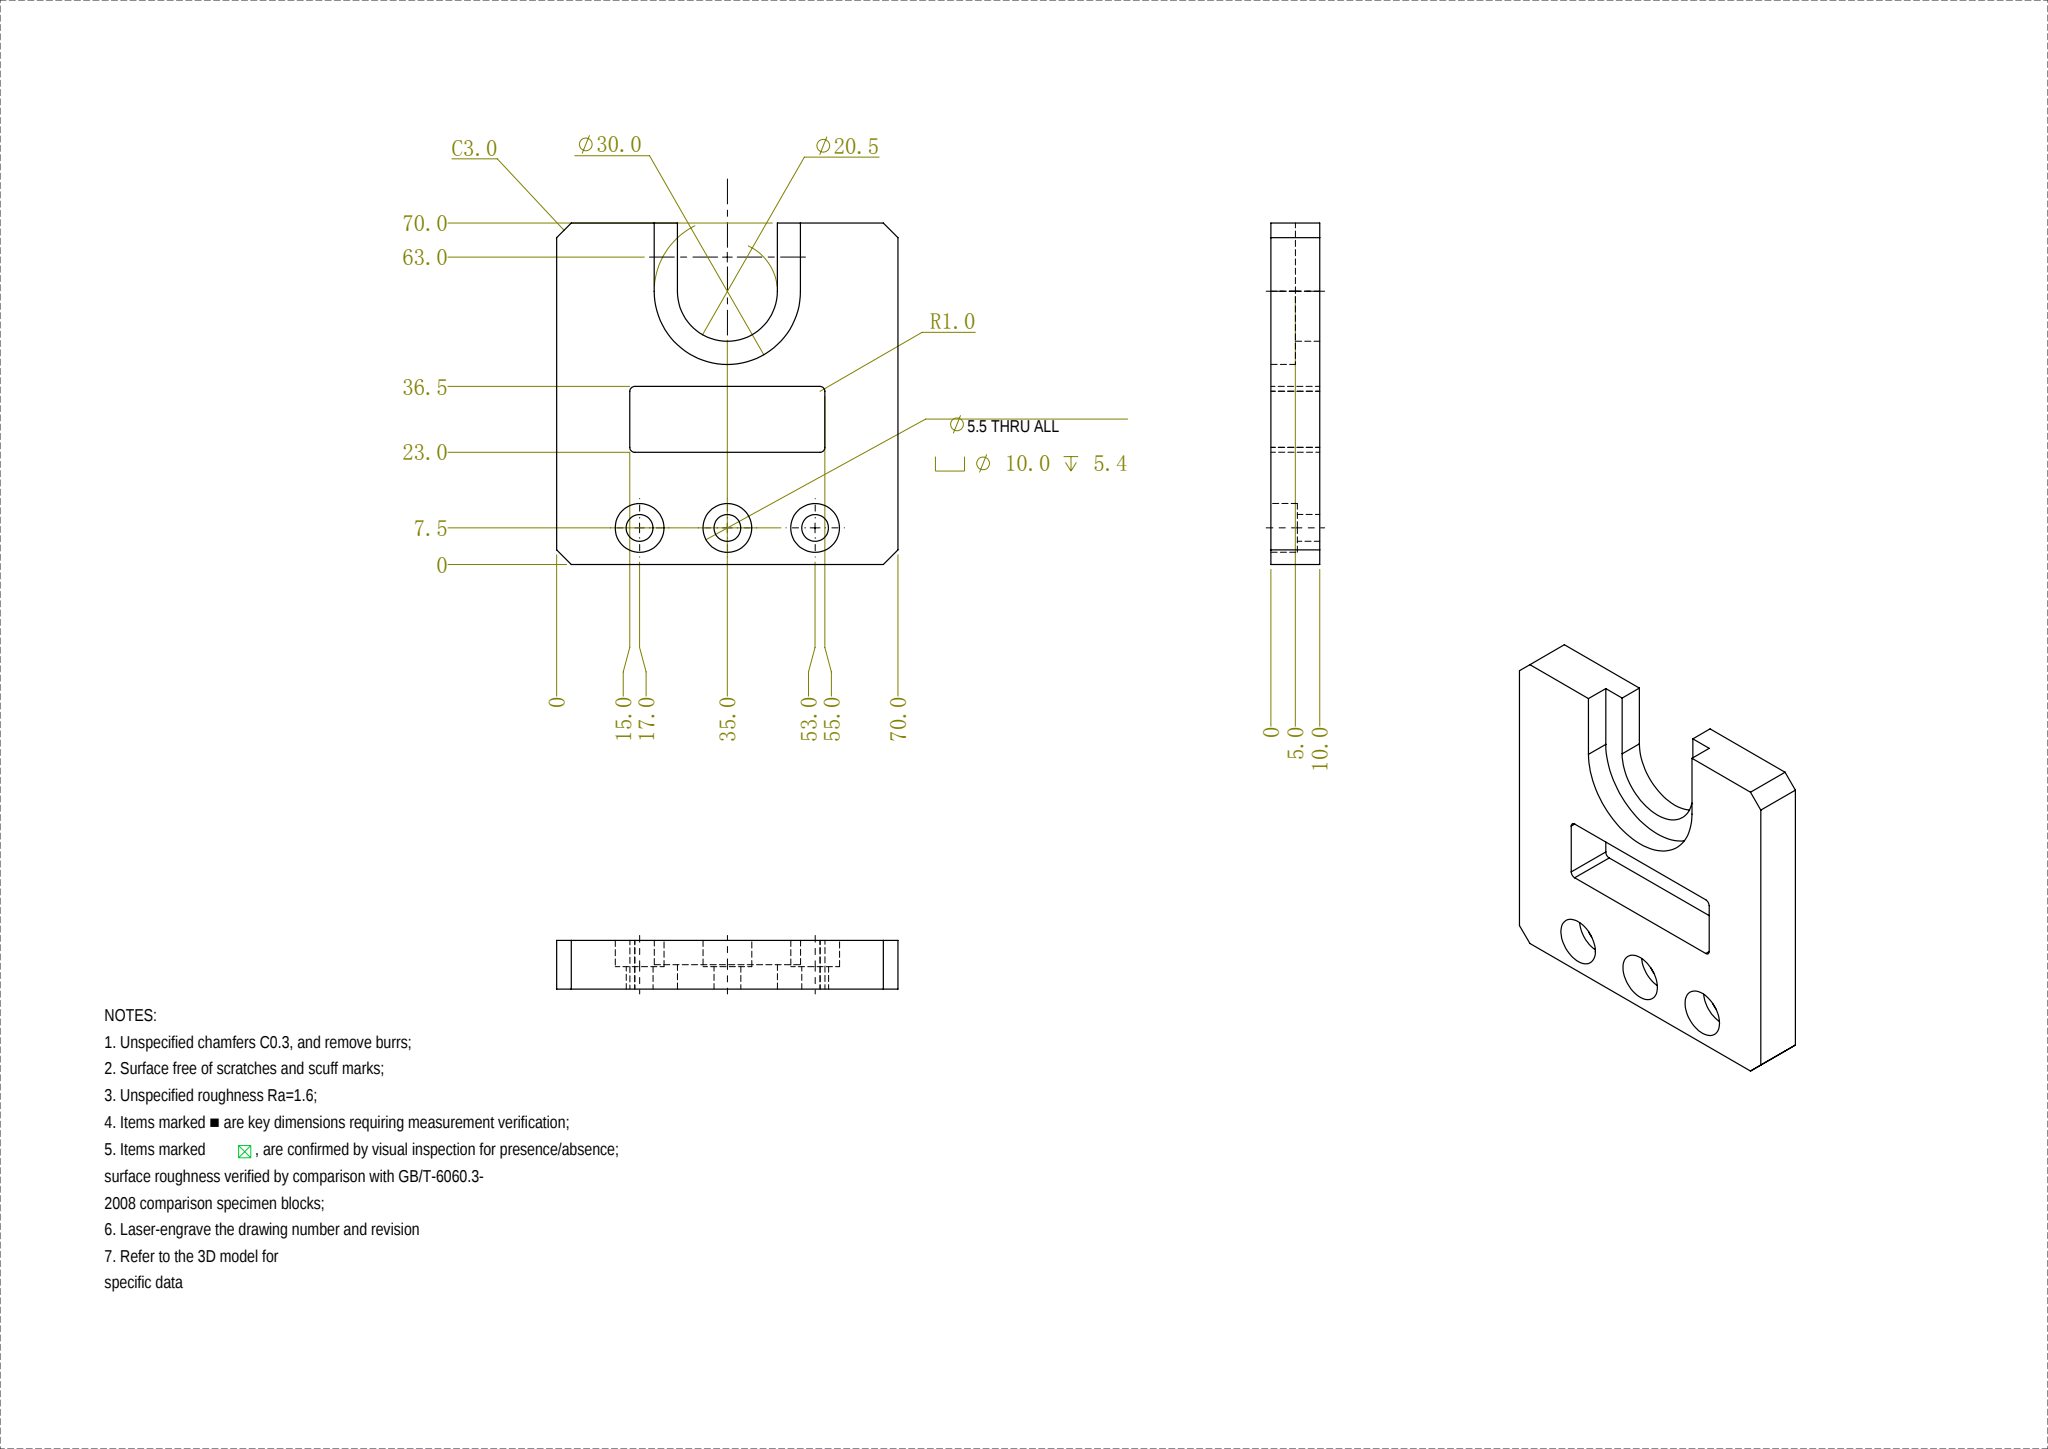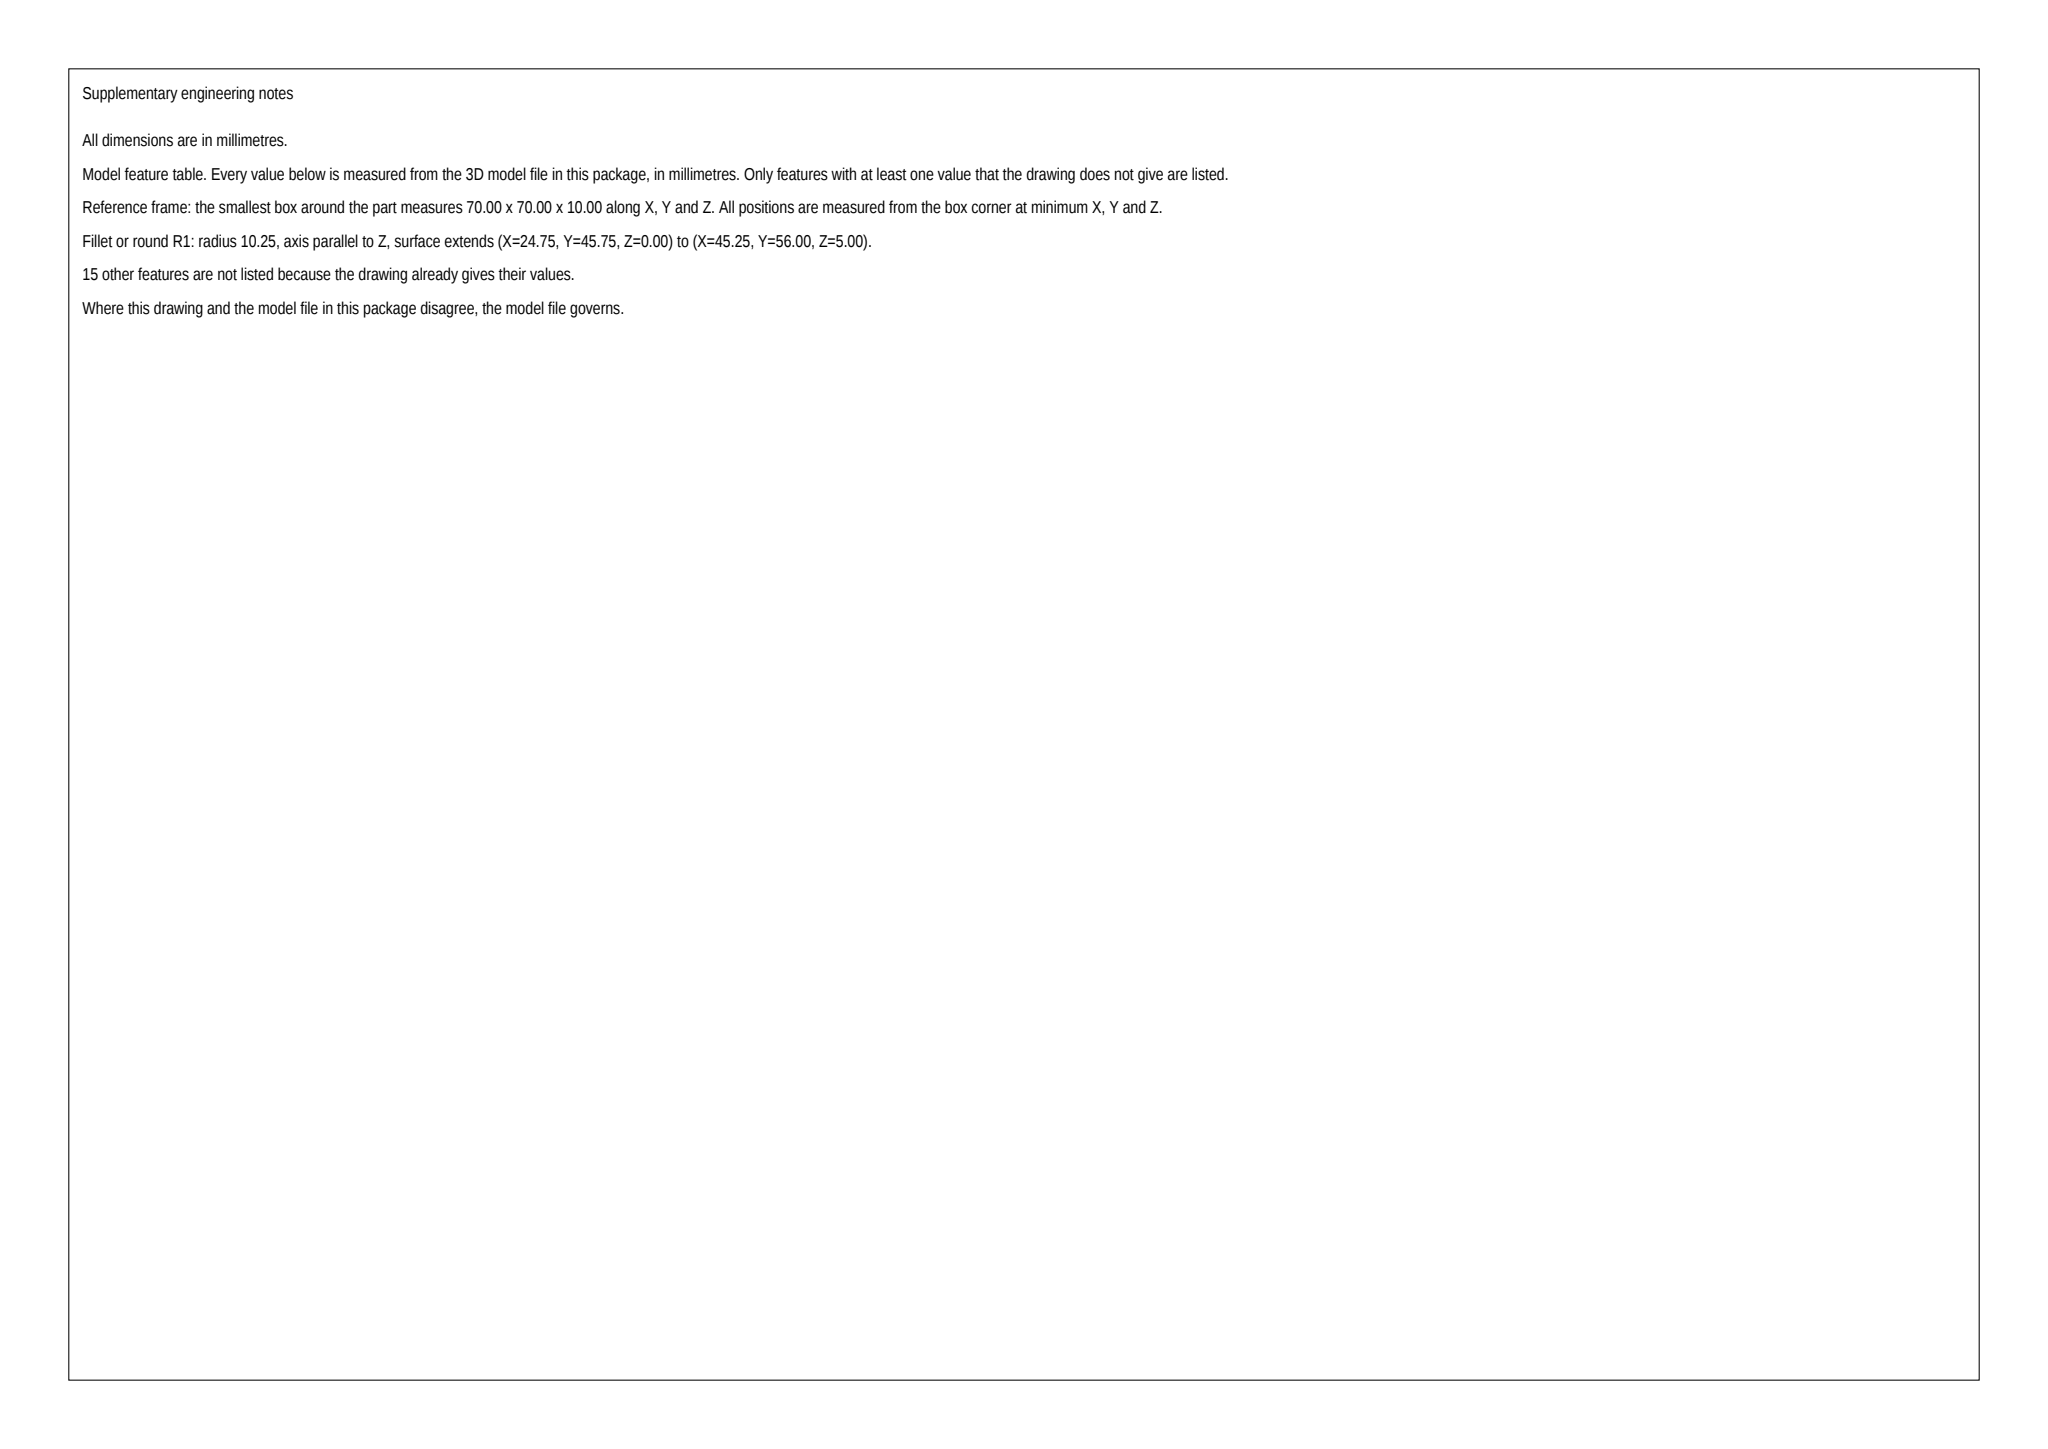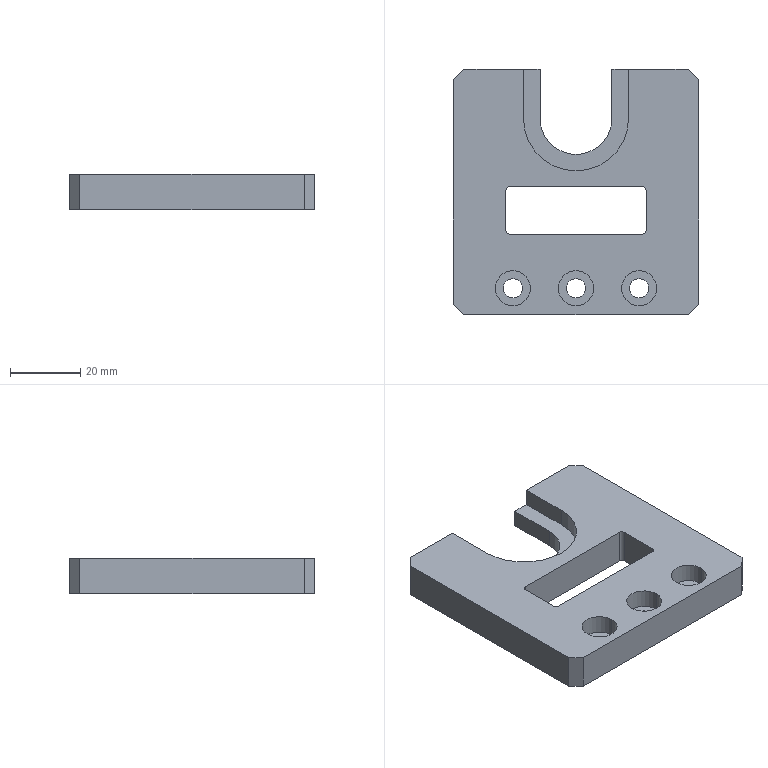Part | SolidWorks | mm | 1 solid | 41 faces | box 70 x 70 x 10 mm | volume 35701 mm3 | plane 23 | cylinder 18 | commonest cylinder face diameters 10 x6 5.5 x6 2 x4 20.5 x1 30 x1
Drawing notes:
U-SLOT STEP: Ø30.0 DP 5.0 FROM FRONT FACE, Ø20.5 THRU REM 5.0, CTR X35.0 Y56.0 | from the solid: Ø30.0 z-cyl len 5.0 & Ø20.5 z-cyl len 5.0 at (35.0,56.0); z-planes 5.0/10.0; x-planes 20.0/50.0 and 24.75/45.25 = slot walls
RECT POCKET 40.0 W X 13.5 H, R1.0 CNRS, THRU ALL, SYM ABT CL X35.0 | from the solid: x-planes 15.0/55.0 (40 wide), y-planes 23.0/36.5 (13.5 high); R1 corner cyls Ø2.0 at (16,24)(16,35.5)(54,24)(54,35.5) len 10.0 = full thk
3X Ø5.5 THRU, CBORE Ø10.0 DP 5.4 FROM FRONT FACE, Y7.5, X17.0/35.0/53.0 | from the solid: Ø5.5 len 4.6 + Ø10.0 len 5.4 = 10.0 thk at (17,7.5),(35,7.5),(53,7.5); z-plane 4.6 (3X) = cbore floors; 18.0 pitch
C3.0 CHAMFER 4X AT CORNERS OF 70.0 X 70.0 OUTLINE | from the solid: bbox 70.0x70.0x10.0; outline planes x=0/70, y=0/70 with 4 corner chamfers in front view/iso
build123d program:
from build123d import *

# Parameters (mm, degrees)
SKETCH1_W                                       = 70
SKETCH1_H                                       = 70
BOSS_EXTRUDE1_DEPTH                             = 5
CUT_EXTRUDE1_DEPTH                              = 51.498
CUT_EXTRUDE2_DEPTH                              = 5
M5_HEX_SOCKET_HEAD_CAP_SCREW_CBORE1_D           = 5.5
M5_HEX_SOCKET_HEAD_CAP_SCREW_CBORE1_CBORE_D     = 10
M5_HEX_SOCKET_HEAD_CAP_SCREW_CBORE1_CBORE_DEPTH = 5.4
CHAMFER1_SIZE                                   = 3
SKETCH6_W                                       = 40
SKETCH6_H                                       = 13.5
CUT_EXTRUDE3_DEPTH                              = 51.498
FILLET1_R                                       = 1


with BuildPart() as part:
    # Sketch1 → Boss-Extrude1 (new, symmetric)
    with BuildSketch(Plane.XY):
        Rectangle(SKETCH1_W, SKETCH1_H)
    extrude(amount=BOSS_EXTRUDE1_DEPTH, both=True)

    # Sketch2 → Cut-Extrude1 (cut, through all)
    with BuildSketch(Plane.XY.offset(5)):
        with BuildLine():
            Line((10.25, 35), (10.25, 21))
            ThreePointArc((10.25, 21), (0, 10.75), (-10.25, 21))
            Line((-10.25, 21), (-10.25, 35))
            ThreePointArc((-10.25, 35), (0, 45.25), (10.25, 35))
        make_face()
    extrude(amount=-CUT_EXTRUDE1_DEPTH, mode=Mode.SUBTRACT)

    # Sketch3 → Cut-Extrude2 (cut)
    with BuildSketch(Plane.XY.offset(5)):
        with BuildLine():
            Line((-15, 21), (-15, 35))
            ThreePointArc((-15, 35), (0, 50), (15, 35))
            Line((15, 35), (15, 21))
            ThreePointArc((15, 21), (0, 6), (-15, 21))
        make_face()
    extrude(amount=-CUT_EXTRUDE2_DEPTH, mode=Mode.SUBTRACT)

    # M5 Hex Socket Head Cap Screw CBORE1 (through all)
    with Locations(Plane.XY.offset(5)):
        with Locations((-18, -27.5), (0, -27.5), (18, -27.5)):
            CounterBoreHole(M5_HEX_SOCKET_HEAD_CAP_SCREW_CBORE1_D / 2, M5_HEX_SOCKET_HEAD_CAP_SCREW_CBORE1_CBORE_D / 2, M5_HEX_SOCKET_HEAD_CAP_SCREW_CBORE1_CBORE_DEPTH)

    # Chamfer1
    chamfer1_edges = [part.edges().sort_by_distance(p)[0] for p in [
        (35, -35, 0),
        (-35, -35, 0),
        (-35, 35, 0),
        (35, 35, 0),
    ]]
    chamfer(chamfer1_edges, length=CHAMFER1_SIZE)

    # Sketch6 → Cut-Extrude3 (cut, through all)
    with BuildSketch(Plane(origin=(0, 0, -5), x_dir=(-1, 0, 0), z_dir=(0, 0, -1))):
        with Locations((0, -5.25)):
            Rectangle(SKETCH6_W, SKETCH6_H)
    extrude(amount=-CUT_EXTRUDE3_DEPTH, mode=Mode.SUBTRACT)

    # Fillet1
    fillet1_edges = [part.edges().sort_by_distance(p)[0] for p in [
        (20, -12, 0),
        (20, 1.5, 0),
        (-20, 1.5, 0),
        (-20, -12, 0),
    ]]
    fillet(fillet1_edges, radius=FILLET1_R)


solid = part.part